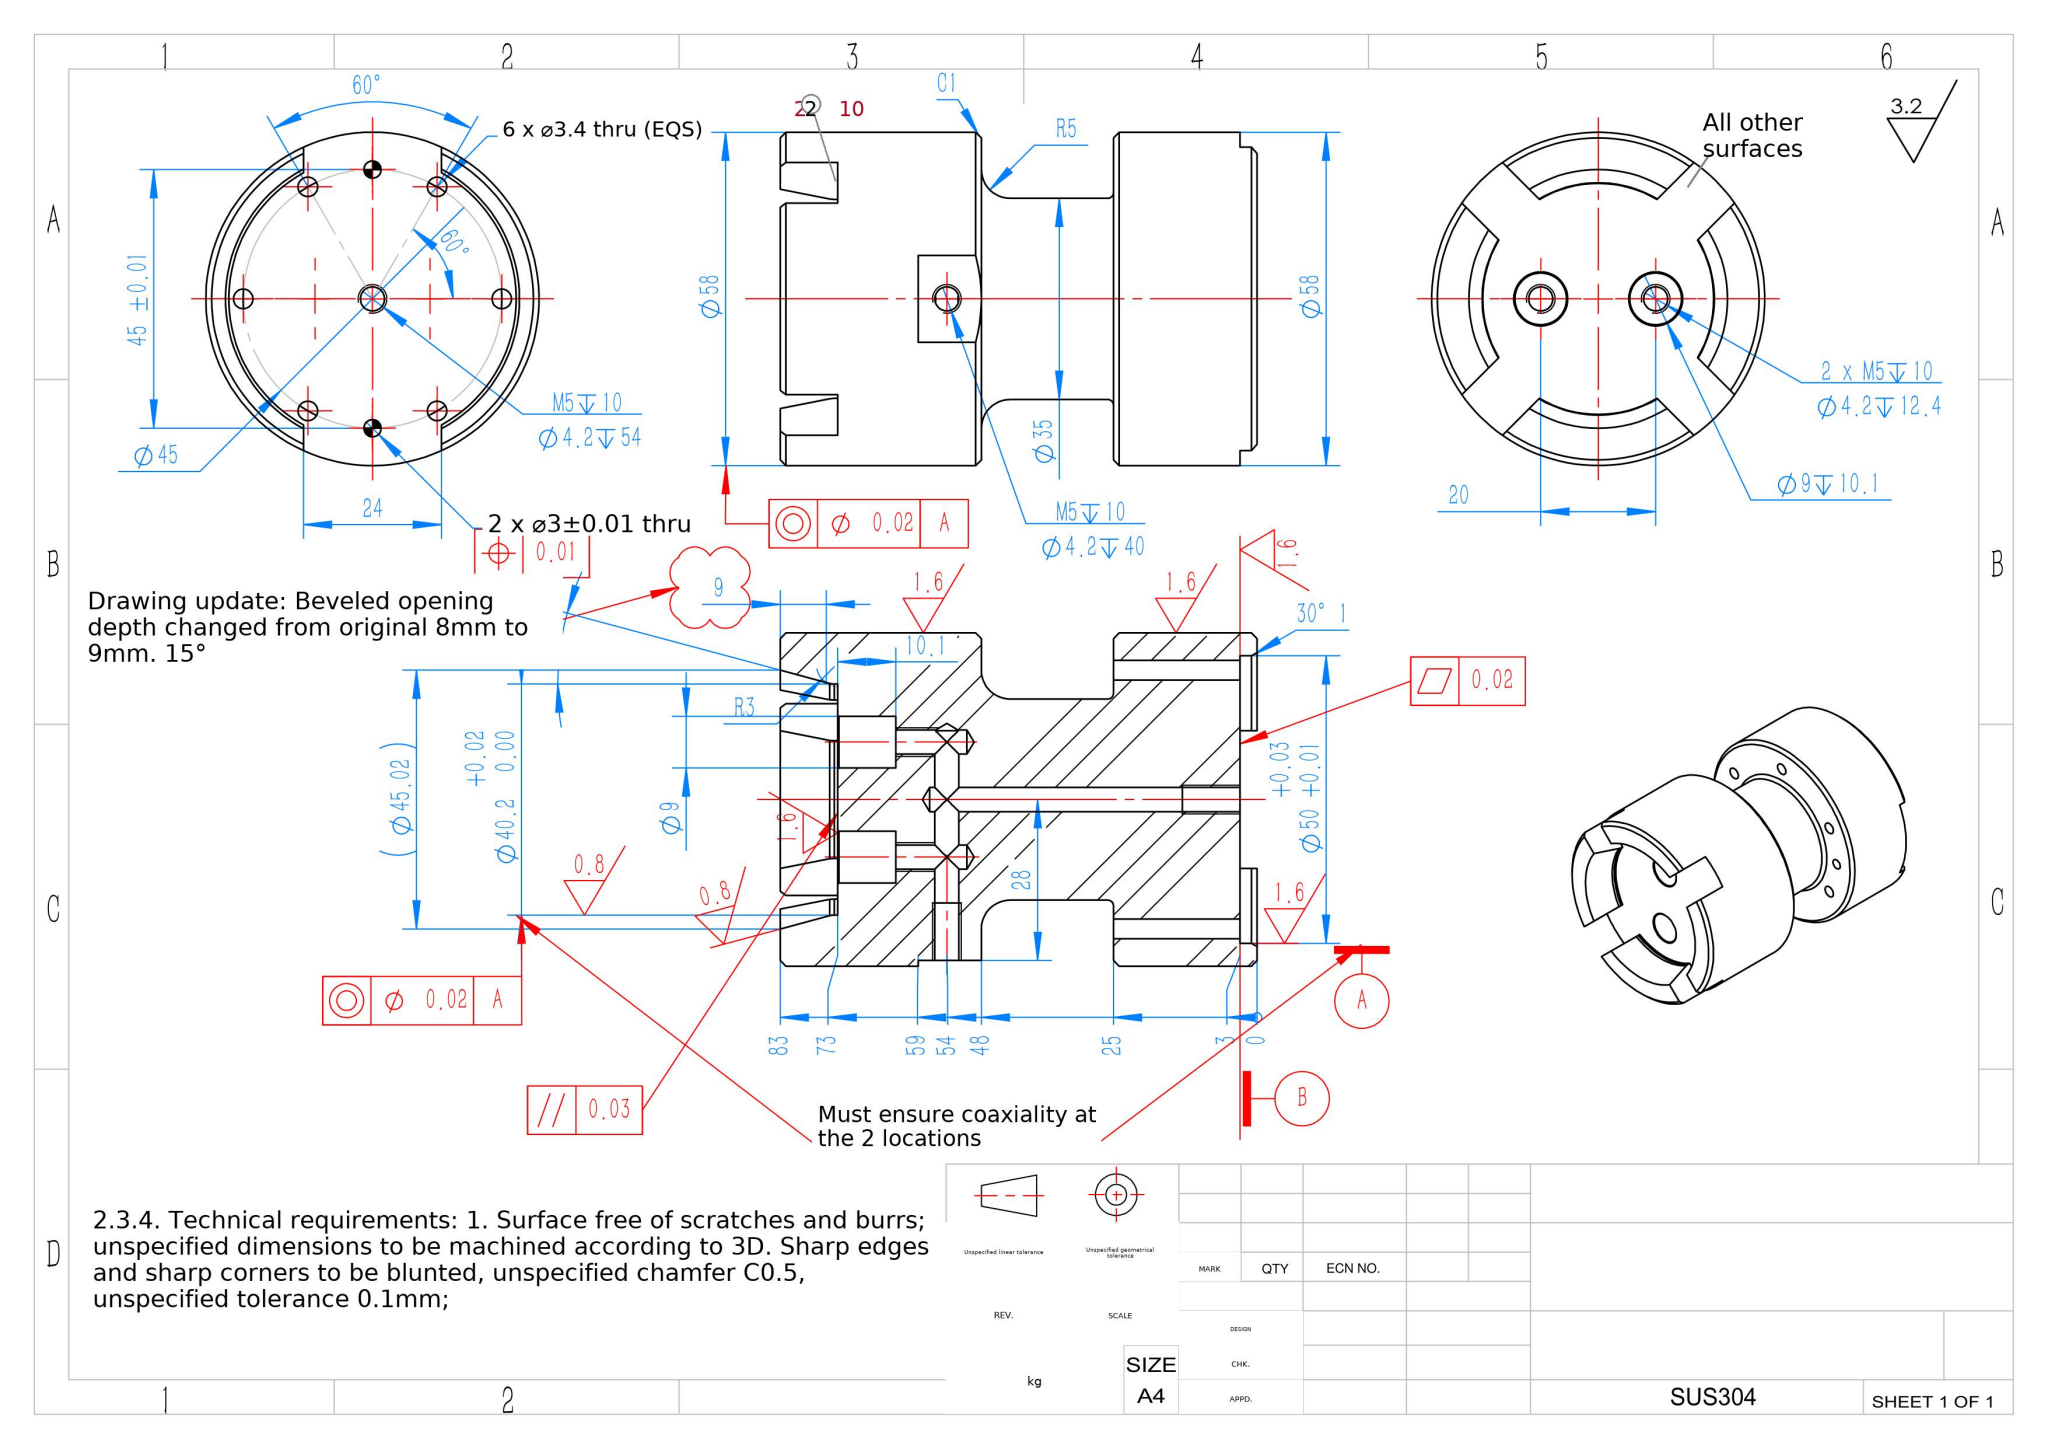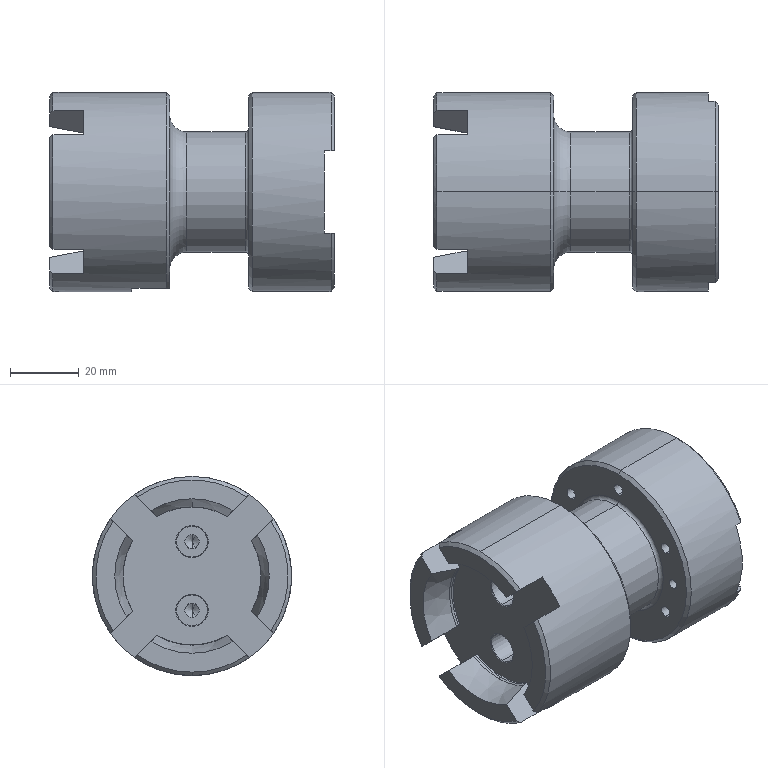Part | SolidWorks | mm | material SUS304 | 1 solid | 121 faces | box 83 x 58 x 58 mm | volume 152783 mm3 | cylinder 54 | cone 32 | plane 26 | torus 9 | commonest cylinder face diameters 4.2 x20 3.4 x12 40.2 x5 9 x4 3 x4 58 x4 50 x3 35 x2
build123d program:
from build123d import *

# Parameters (mm, degrees)
SKETCH2_W                = 23
SKETCH2_H                = 17.5
SKETCH3_R                = 29
BOSS_EXTRUDE1_DEPTH      = 25
SKETCH4_R                = 25
CUT_EXTRUDE1_DEPTH       = 3
M3_TAPPED_HOLE1_D        = 3.4
F_3_0_3_DIAMETER_HOLE1_D = 3
BOSS_EXTRUDE2_START      = 35
SKETCH9_R                = 29
BOSS_EXTRUDE2_DEPTH      = 35
SKETCH10_R               = 20.1
CUT_EXTRUDE2_DEPTH       = 10
CHAMFER1_SIZE            = 9
CHAMFER1_SIZE2           = 2.412
CHAMFER2_SIZE            = 1
FILLET1_R                = 3
SKETCH11_W               = 24
SKETCH11_H               = 70
CUT_EXTRUDE3_DEPTH       = 5
CHAMFER3_SIZE            = 1
CHAMFER3_SIZE2           = 0.5774
CHAMFER4_SIZE            = 1
CHAMFER4_SIZE2           = 0.5774
SKETCH14_R               = 4.5
CUT_EXTRUDE5_DEPTH       = 10.1
CHAMFER6_SIZE            = 0.2
M5_TAPPED_HOLE1_D        = 4.2
M5_TAPPED_HOLE1_DEPTH    = 12.4
M5_TAPPED_HOLE1_TIP      = 1.262
M5_TAPPED_HOLE3_D        = 4.2
M5_TAPPED_HOLE3_DEPTH    = 54
M5_TAPPED_HOLE3_TIP      = 1.262
FILLET2_R                = 1
FILLET3_R                = 5
SKETCH23_W               = 14
SKETCH23_H               = 70.544
CUT_EXTRUDE7_DEPTH       = 2
M5_TAPPED_HOLE4_D        = 4.2
M5_TAPPED_HOLE4_DEPTH    = 40
M5_TAPPED_HOLE4_TIP      = 1.262
CUT_EXTRUDE8_DEPTH       = 20
CIRPATTERN1_COUNT        = 4


with BuildPart() as part:
    # Sketch2 → Revolve1 (revolve)
    with BuildSketch(Plane.XY, mode=Mode.PRIVATE) as revolve1_sk:
        with Locations((11.5, 8.75)):
            Rectangle(SKETCH2_W, SKETCH2_H)
    revolve(revolve1_sk.sketch.rotate(Axis((0, 0, 0), (1, 0, 0)), 90), axis=Axis((0, 0, 0), (1, 0, 0)))

    # Sketch3 → Boss-Extrude1 (add)
    with BuildSketch(Plane(origin=(23, 0, 0), x_dir=(0, 0, -1), z_dir=(1, 0, 0))):
        Circle(SKETCH3_R)
    extrude(amount=BOSS_EXTRUDE1_DEPTH)

    # Sketch4 → Cut-Extrude1 (cut)
    with BuildSketch(Plane(origin=(48, 0, 0), x_dir=(0, 0, -1), z_dir=(1, 0, 0))):
        Circle(SKETCH4_R)
    extrude(amount=-CUT_EXTRUDE1_DEPTH, mode=Mode.SUBTRACT)

    # M3 Tapped Hole1 (through all)
    with Locations(Plane.ZY.offset(-23)):
        with Locations((22.5, 0), (11.25, -19.486), (-11.25, -19.486), (-22.5, 0), (-11.25, 19.486), (11.25, 19.486)):
            Hole(M3_TAPPED_HOLE1_D / 2)

    # 3.0 _3_ Diameter Hole1 (through all)
    with Locations(Plane.ZY.offset(-23)):
        with Locations((0, -22.5), (0, 22.5)):
            Hole(F_3_0_3_DIAMETER_HOLE1_D / 2)

    # Sketch9 → Boss-Extrude2 (add)
    with BuildSketch(Plane.ZY.offset(BOSS_EXTRUDE2_START)):
        with Locations(Location((0, 0, 0), (0, 0, 180))):
            Circle(SKETCH9_R)
    extrude(amount=-BOSS_EXTRUDE2_DEPTH)

    # Sketch10 → Cut-Extrude2 (cut)
    with BuildSketch(Plane.ZY.offset(35)):
        Circle(SKETCH10_R)
    extrude(amount=-CUT_EXTRUDE2_DEPTH, mode=Mode.SUBTRACT)

    # Chamfer1
    chamfer1_edges = [part.edges().sort_by_distance(p)[0] for p in [
        (-35, 0, -20.1),
    ]]
    chamfer1_side = [part.faces().sort_by_distance(p)[0] for p in [
        (-30, 0, -20.1),
    ]]
    chamfer(chamfer1_edges, length=CHAMFER1_SIZE, length2=CHAMFER1_SIZE2, reference=chamfer1_side[0])

    # Chamfer2
    chamfer2_edges = [part.edges().sort_by_distance(p)[0] for p in [
        (0, 0, 29),
        (-35, 0, 29),
        (23, 0, 29),
        (48, 0, 29),
    ]]
    chamfer(chamfer2_edges, length=CHAMFER2_SIZE)

    # Fillet1
    fillet1_edges = [part.edges().sort_by_distance(p)[0] for p in [
        (-26, 0, -20.1),
    ]]
    fillet(fillet1_edges, radius=FILLET1_R)

    # Sketch11 → Cut-Extrude3 (cut)
    with BuildSketch(Plane(origin=(45, 0, 0), x_dir=(0, 0, -1), z_dir=(1, 0, 0))):
        Rectangle(SKETCH11_W, SKETCH11_H)
    extrude(amount=CUT_EXTRUDE3_DEPTH, mode=Mode.SUBTRACT)

    # Chamfer3
    chamfer3_edges = [part.edges().sort_by_distance(p)[0] for p in [
        (48, 0, -25),
    ]]
    chamfer3_side = [part.faces().sort_by_distance(p)[0] for p in [
        (46.5, 0, -25),
    ]]
    chamfer(chamfer3_edges, length=CHAMFER3_SIZE, length2=CHAMFER3_SIZE2, reference=chamfer3_side[0])

    # Chamfer4
    chamfer4_edges = [part.edges().sort_by_distance(p)[0] for p in [
        (48, 0, 25),
    ]]
    chamfer4_side = [part.faces().sort_by_distance(p)[0] for p in [
        (46.5, 0, 25),
    ]]
    chamfer(chamfer4_edges, length=CHAMFER4_SIZE, length2=CHAMFER4_SIZE2, reference=chamfer4_side[0])

    # Sketch14 → Cut-Extrude5 (cut)
    with BuildSketch(Plane.ZY.offset(25)):
        with Locations((10, 0)):
            Circle(SKETCH14_R)
        with Locations((-10, 0)):
            Circle(SKETCH14_R)
    extrude(amount=-CUT_EXTRUDE5_DEPTH, mode=Mode.SUBTRACT)

    # Chamfer6
    chamfer6_edges = [part.edges().sort_by_distance(p)[0] for p in [
        (-25, 0, 5.5),
        (-25, 0, -14.5),
    ]]
    chamfer(chamfer6_edges, length=CHAMFER6_SIZE)

    # M5 Tapped Hole1
    with Locations(Plane.ZY.offset(14.9)):
        with Locations((10, 0), (-10, 0)):
            Hole(M5_TAPPED_HOLE1_D / 2, depth=M5_TAPPED_HOLE1_DEPTH)
            with Locations((0, 0, -(M5_TAPPED_HOLE1_DEPTH + M5_TAPPED_HOLE1_TIP / 2))):  # 118° drill point
                Cone(0, M5_TAPPED_HOLE1_D / 2, M5_TAPPED_HOLE1_TIP, mode=Mode.SUBTRACT)

    # M5 Tapped Hole3
    with Locations(Plane(origin=(45, 0, 0), x_dir=(0, 0, -1), z_dir=(1, 0, 0))):
        with Locations((0, 0)):
            Hole(M5_TAPPED_HOLE3_D / 2, depth=M5_TAPPED_HOLE3_DEPTH)
            with Locations((0, 0, -(M5_TAPPED_HOLE3_DEPTH + M5_TAPPED_HOLE3_TIP / 2))):  # 118° drill point
                Cone(0, M5_TAPPED_HOLE3_D / 2, M5_TAPPED_HOLE3_TIP, mode=Mode.SUBTRACT)

    # Fillet2
    fillet2_edges = [part.edges().sort_by_distance(p)[0] for p in [
        (23, 0, -17.5),
    ]]
    fillet(fillet2_edges, radius=FILLET2_R)

    # Fillet3
    fillet3_edges = [part.edges().sort_by_distance(p)[0] for p in [
        (0, 0, -17.5),
    ]]
    fillet(fillet3_edges, radius=FILLET3_R)

    # Sketch23 → Cut-Extrude7 (cut)
    with BuildSketch(Plane.XY.offset(-28)):
        with Locations((-4, 0)):
            Rectangle(SKETCH23_W, SKETCH23_H)
    extrude(amount=-CUT_EXTRUDE7_DEPTH, mode=Mode.SUBTRACT)

    # M5 Tapped Hole4
    with Locations(Plane(origin=(0, 0, -28), x_dir=(-1, 0, 0), z_dir=(0, 0, -1))):
        with Locations((6, 0)):
            Hole(M5_TAPPED_HOLE4_D / 2, depth=M5_TAPPED_HOLE4_DEPTH)
            with Locations((0, 0, -(M5_TAPPED_HOLE4_DEPTH + M5_TAPPED_HOLE4_TIP / 2))):  # 118° drill point
                Cone(0, M5_TAPPED_HOLE4_D / 2, M5_TAPPED_HOLE4_TIP, mode=Mode.SUBTRACT)

    # Sketch26 → Cut-Extrude8 (cut)
    with BuildSketch(Plane.ZY.offset(25)):
        Polygon((-26.87, 19.799), (-19.799, 26.87), (-8.485, 15.556), (-15.556, 8.485), align=None)
    cut_extrude8 = extrude(amount=CUT_EXTRUDE8_DEPTH, mode=Mode.SUBTRACT)

    # CirPattern1: Cut-Extrude8 ×4 about axis
    cirpattern1_axis = Axis((0, 0, 0), (1, 0, 0))
    for i in range(1, CIRPATTERN1_COUNT):
        add(cut_extrude8.rotate(cirpattern1_axis, i * 360 / CIRPATTERN1_COUNT), mode=Mode.SUBTRACT)


solid = part.part